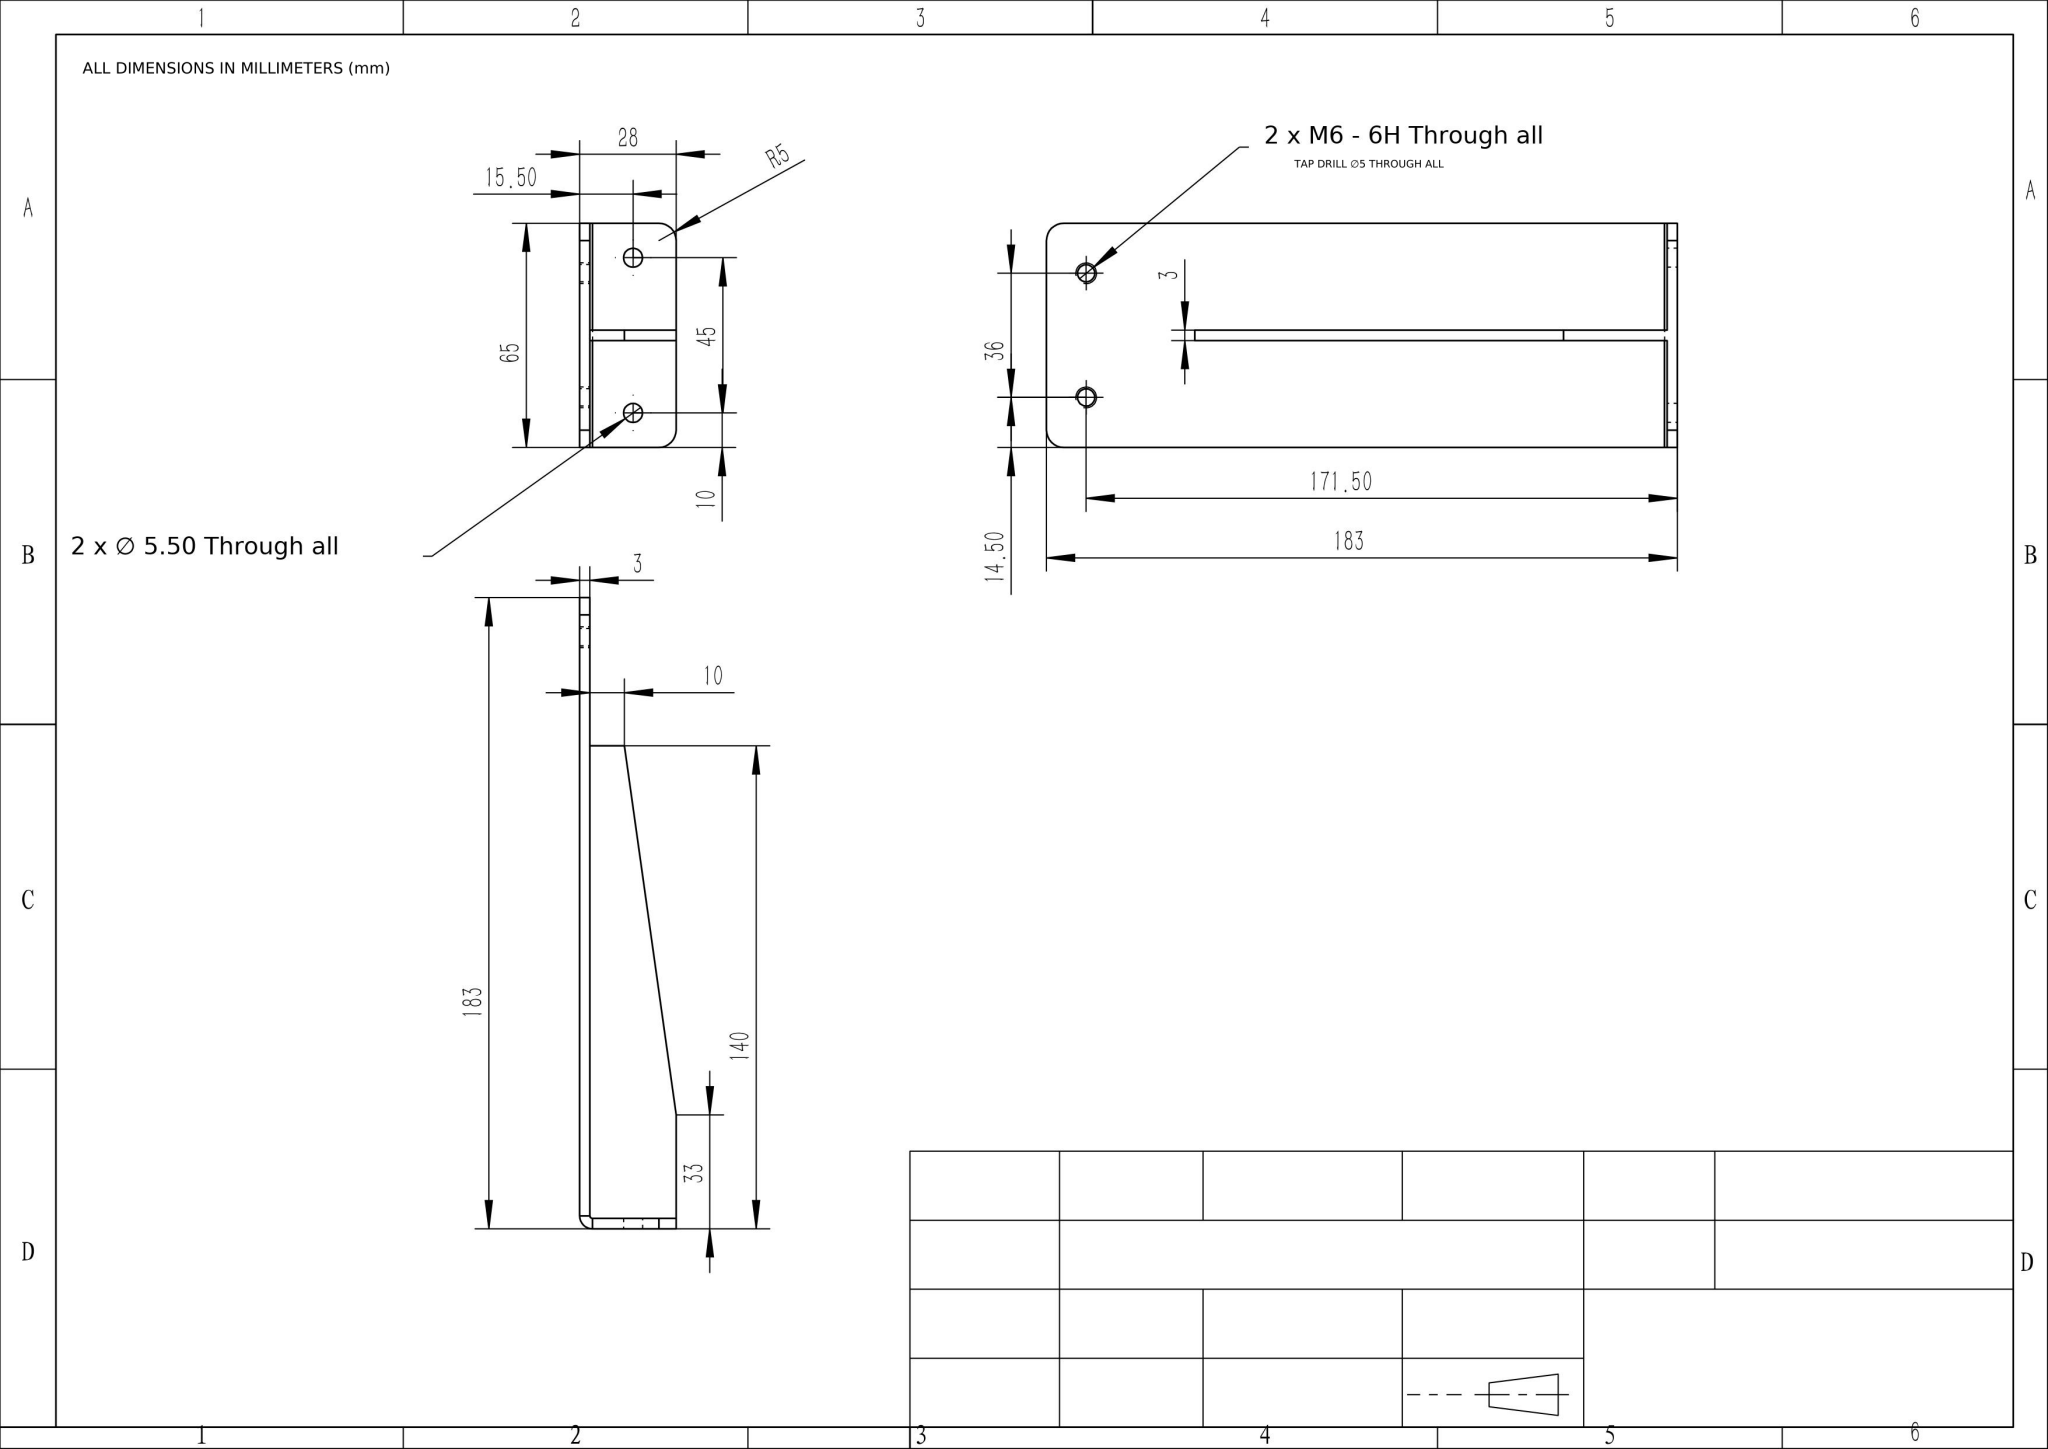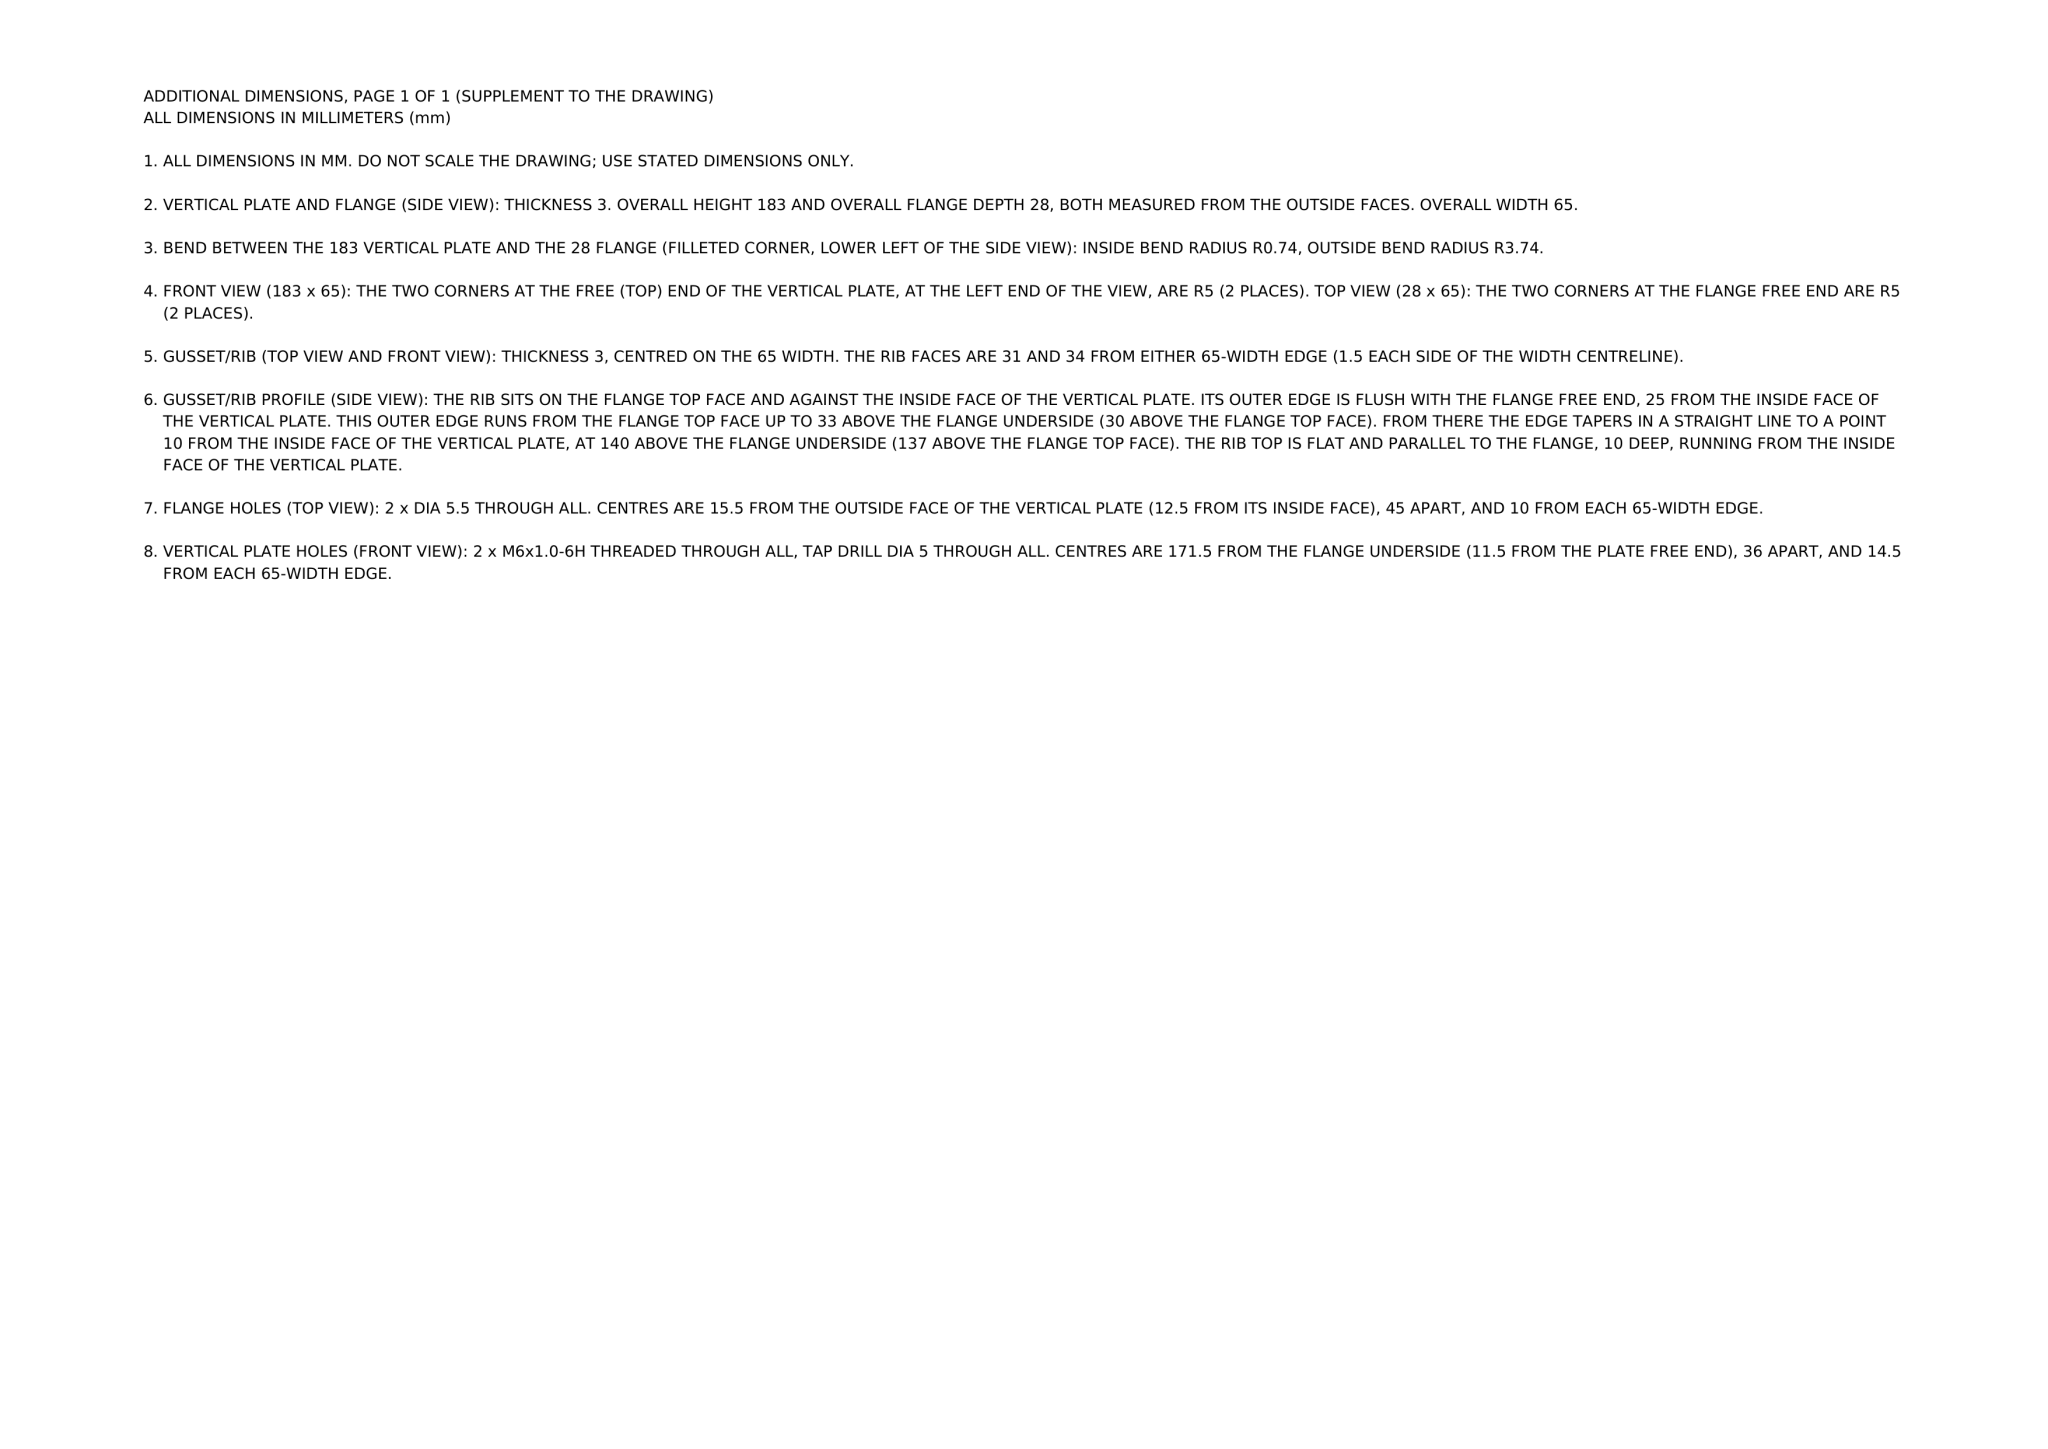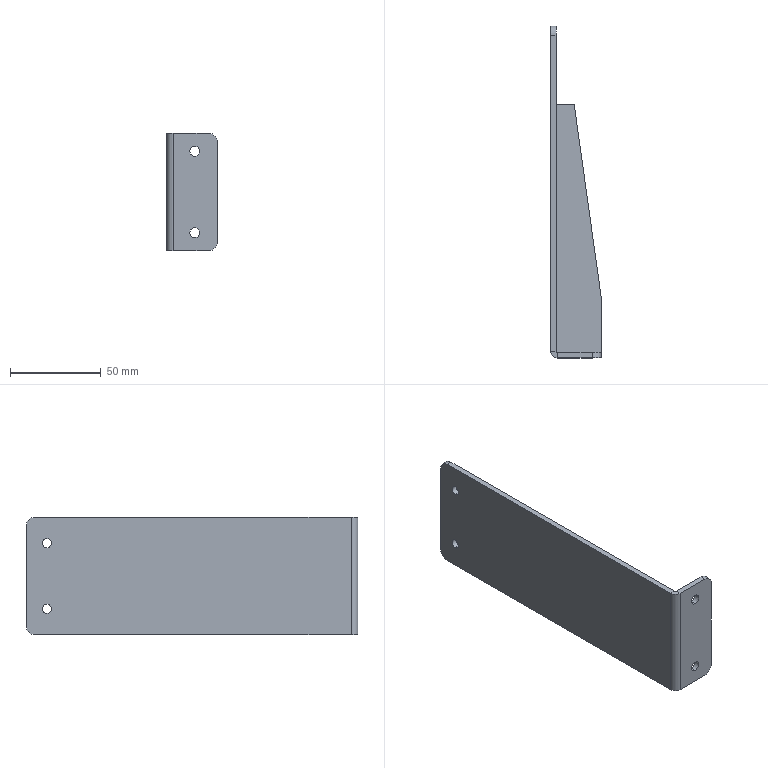Part | NX | mm | 1 solid | 32 faces | box 28 x 183 x 65 mm | volume 47915 mm3 | plane 17 | cylinder 15 | commonest cylinder face diameters 5 x4 5.5 x4 10 x4 1.473 x2 7.473 x1